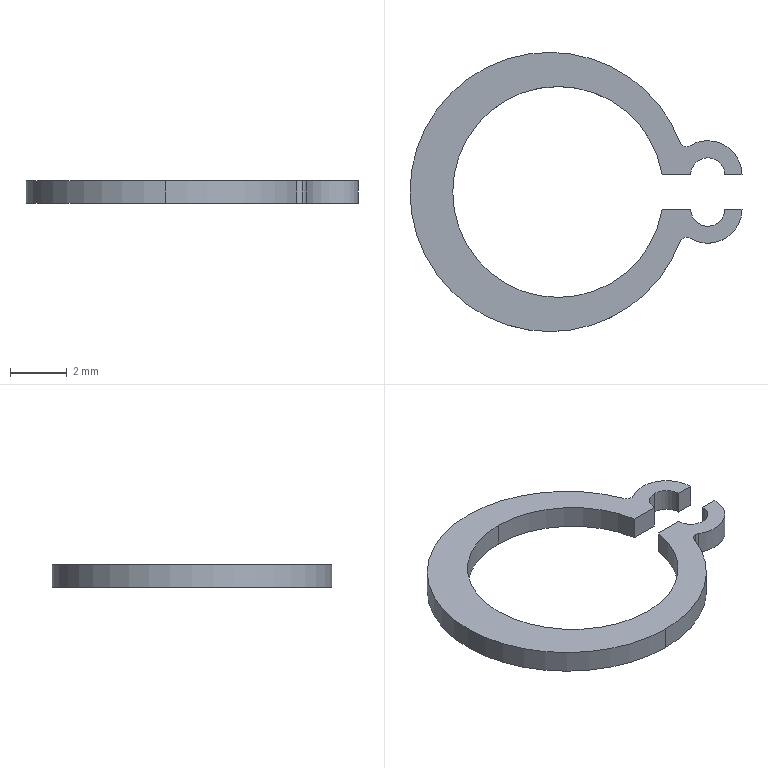Component | SolidWorks | JL001-03-03-1_GB_T894-2017[AxisElasticRetainingRingTypeA(d0_9)8]-1 | 1 solid | 21 faces | box 11.65 x 9.8 x 0.8 mm | volume 27 mm3 | cylinder 15 | plane 6 | commonest cylinder face diameters 9.8 x3 0.48 x3 7.4 x3 1.2 x3 2.4 x3
build123d program:
from build123d import *

# Parameters (mm, degrees)
EXTRUDE1_DEPTH = 0.8


with BuildPart() as part:
    # Dimension Sketch → Extrude1 (new body)
    with BuildSketch(Plane.XY):
        with BuildLine():
            Line((-0.6, -3.651), (-0.6, -4.651))
            ThreePointArc((-0.6, -4.651), (-1.2, -5.251), (-0.6, -5.851))
            Line((-0.6, -5.851), (-0.6, -6.451))
            ThreePointArc((-0.6, -6.451), (-1.646, -5.839), (-1.625, -4.628))
            ThreePointArc((-1.625, -4.628), (-1.603, -4.425), (-1.745, -4.279))
            ThreePointArc((-1.745, -4.279), (0, 5.2), (1.745, -4.279))
            ThreePointArc((1.745, -4.279), (1.603, -4.425), (1.625, -4.628))
            ThreePointArc((1.625, -4.628), (1.646, -5.839), (0.6, -6.451))
            Line((0.6, -6.451), (0.6, -5.851))
            ThreePointArc((0.6, -5.851), (1.2, -5.251), (0.6, -4.651))
            Line((0.6, -4.651), (0.6, -3.651))
            ThreePointArc((0.6, -3.651), (0, 3.7), (-0.6, -3.651))
        make_face()
    extrude(amount=EXTRUDE1_DEPTH)


solid = part.part

# Placed as in the assembly
solid = solid.moved(Location((15, 27.5, 53.5), (0, 0, 90)))